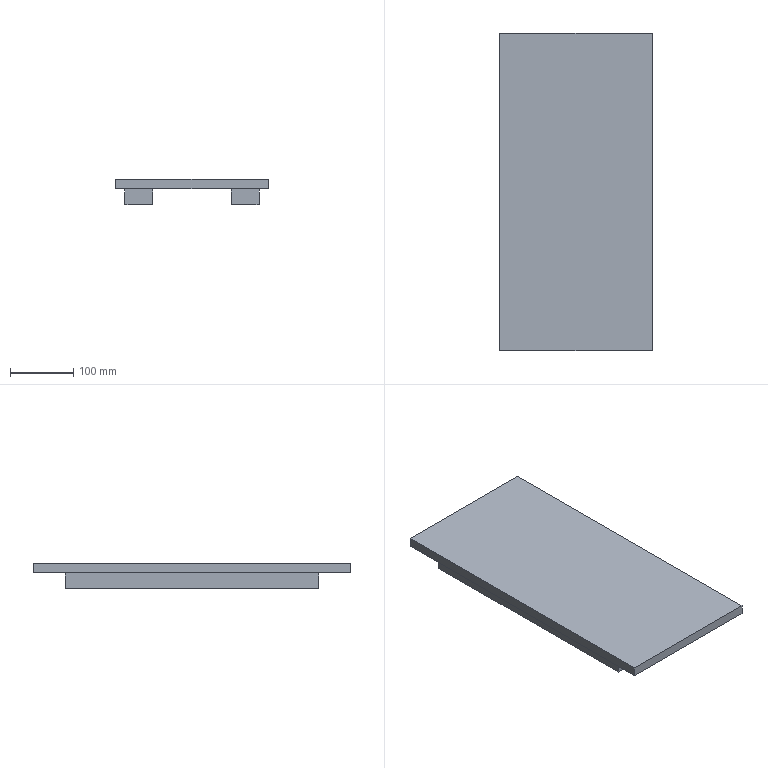CAM job | NX | mm | 3-axis | 2 set-ups | 6 operations | part box 240 x 500 x 40
set-up 1
1. Cavity Milling | Mill Mill5 D50 | CAVITY_MILL | path 59354.965 mm | 230.678 min
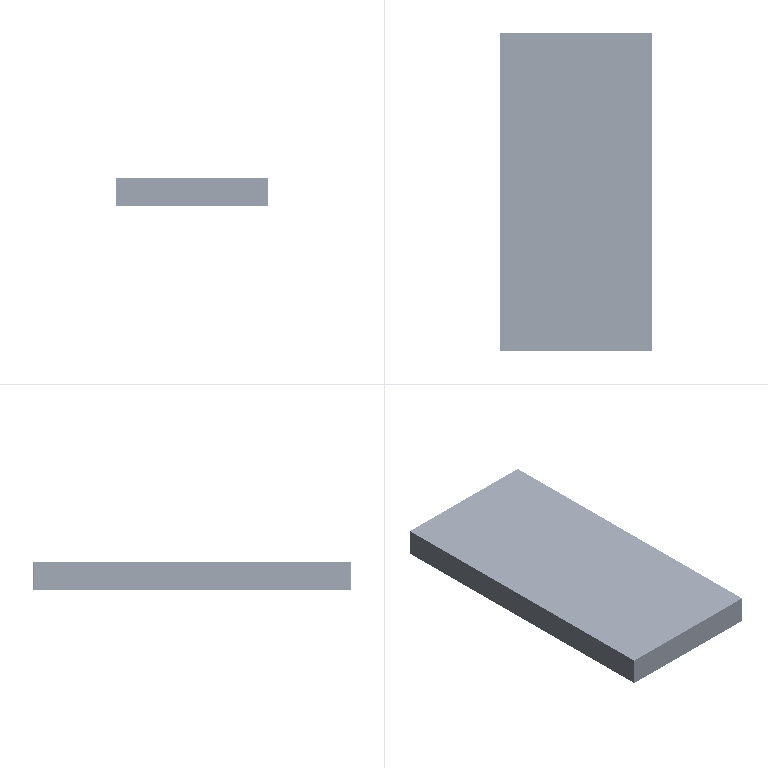2. Volume Based 2.5D Milling | Mill Mill5 D50 | FLOOR_WALL | path 5751.997 mm | 22.93 min
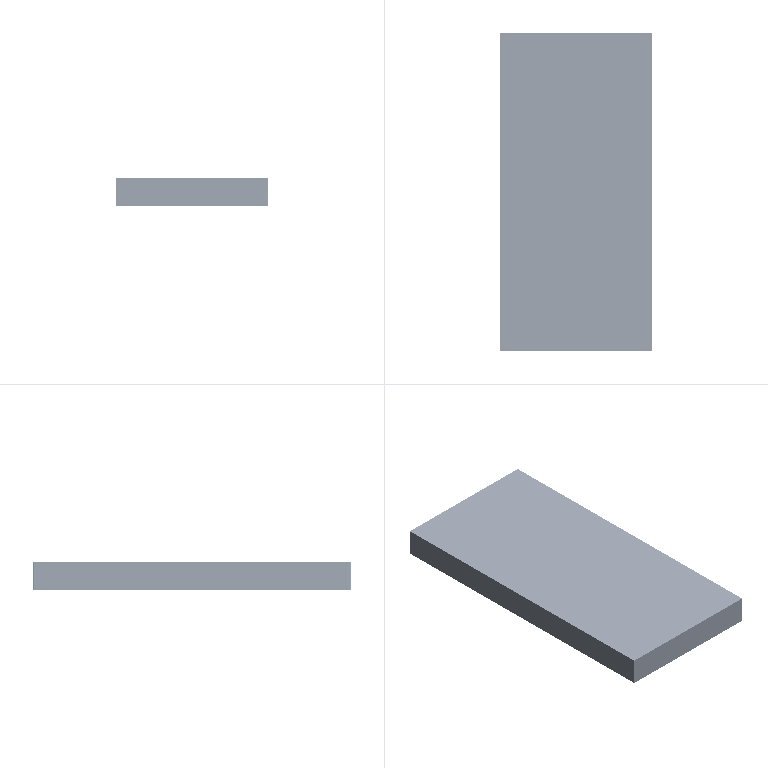3. Cavity Milling | Mill Mill5 D50 | CAVITY_MILL_COPY | path 37785.363 mm | 149.73 min
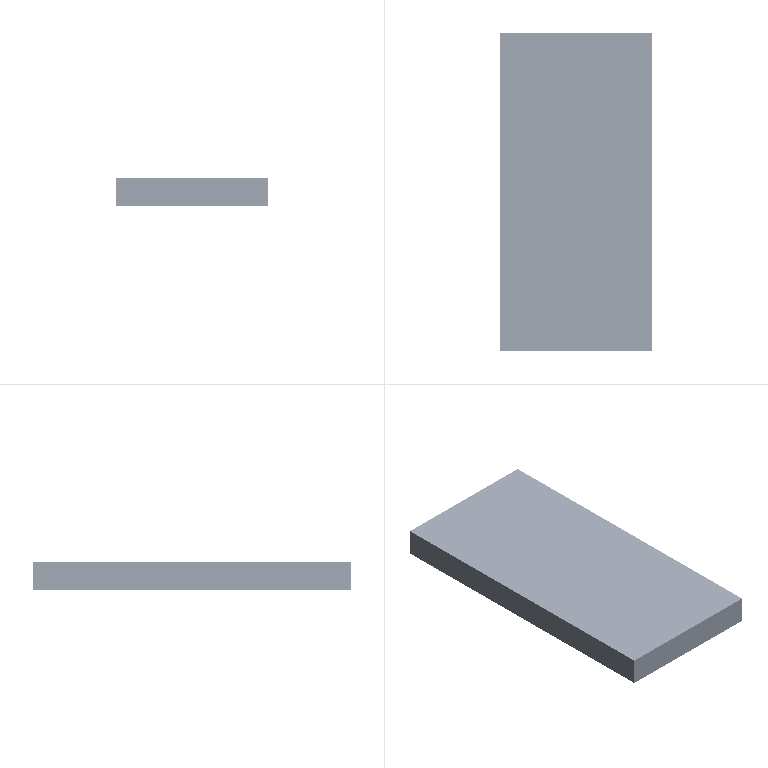set-up 2
4. Cavity Milling | Mill Mill5 D50 | CAVITY_MILL_COPY_1 | path 144060.415 mm | 428.57 min
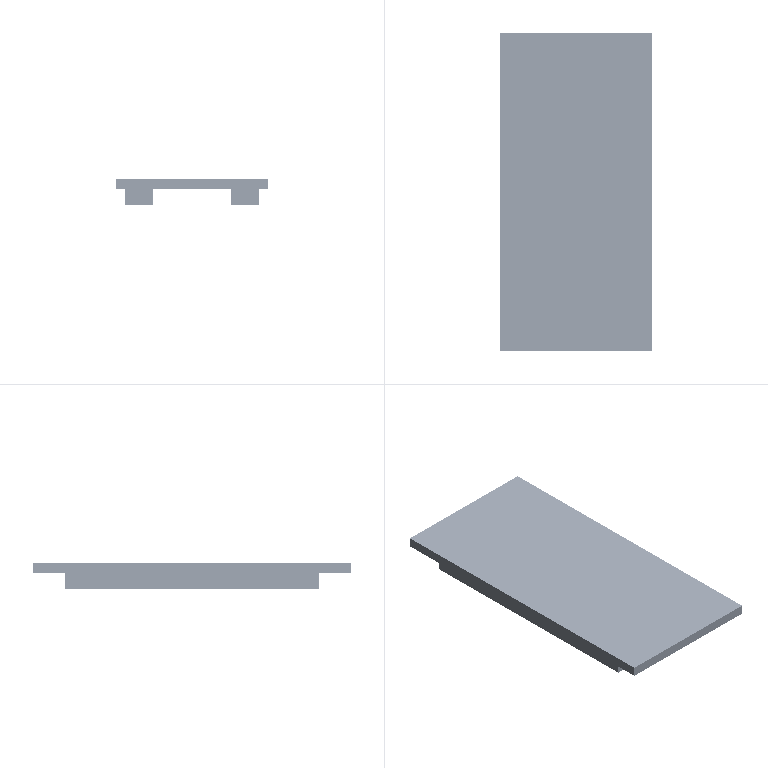5. Volume Based 2.5D Milling | Mill Mill5 D21 | FLOOR_WALL_COPY | path 16489.25 mm | 63.535 min
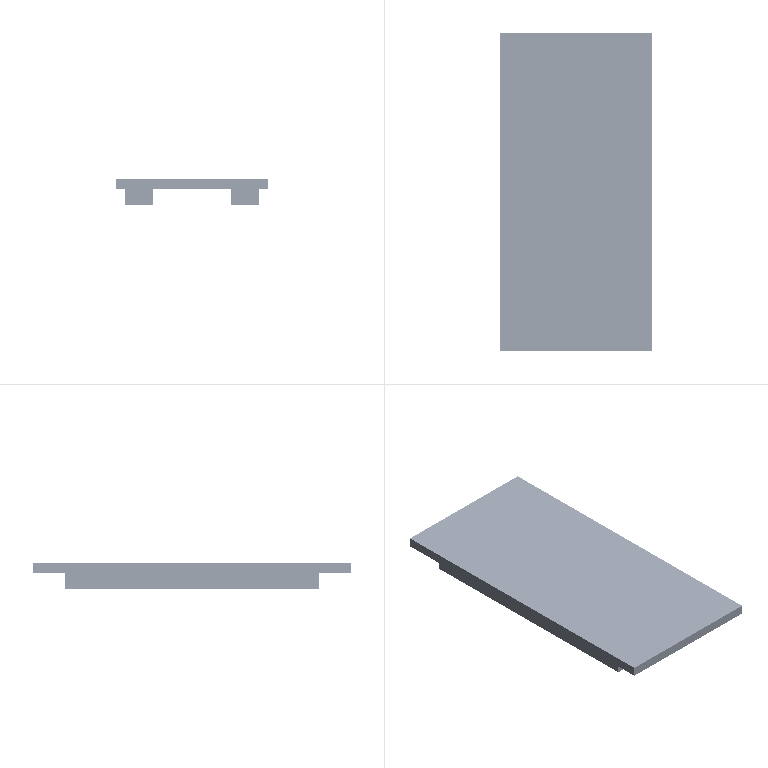6. Volume Based 2.5D Milling | Mill Mill5 D21 | FLOOR_WALL_COPY_COPY | path 33302.637 mm | 108.52 min